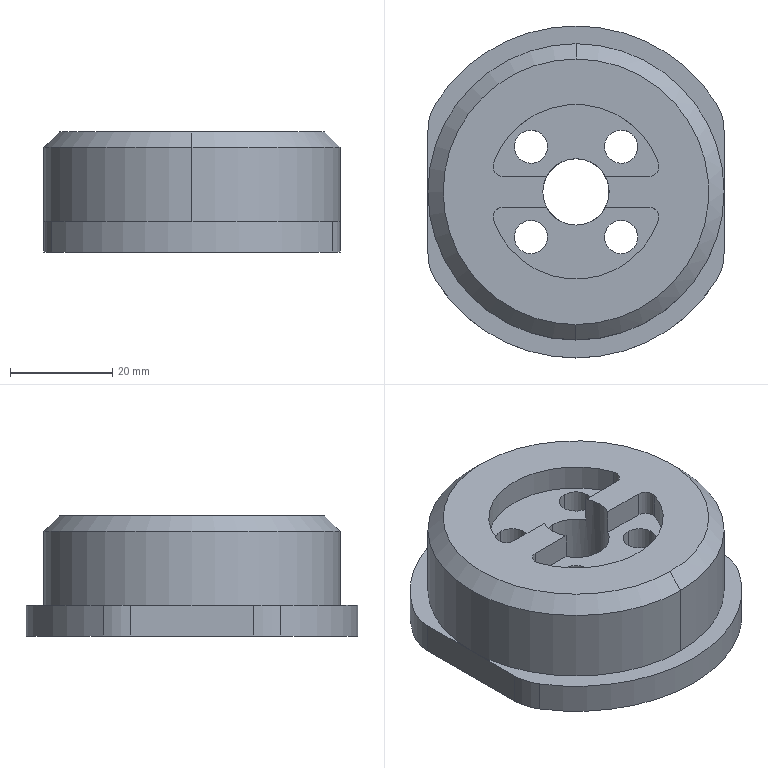CAM job | Mastercam | mm | 9 operations | part box 58 x 65 x 23.5
1. Contour (Ramp) | 9 - 10 平铣刀
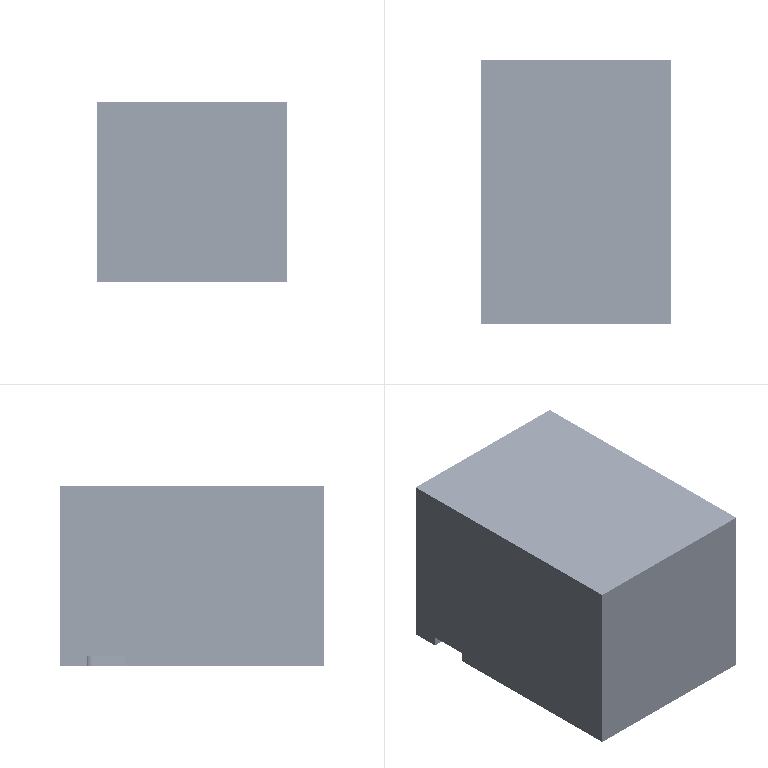2. Contour (2D) | 10 - 10 平铣刀
3. Drill/Counterbore | 7 - 6 倒角刀
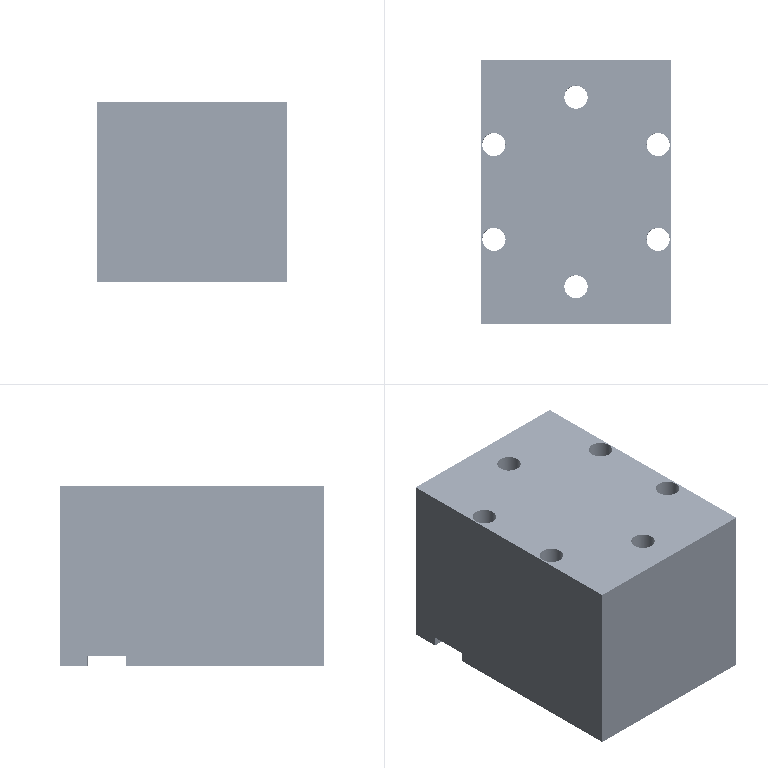4. Contour (Ramp) | 6 - 6 平铣刀
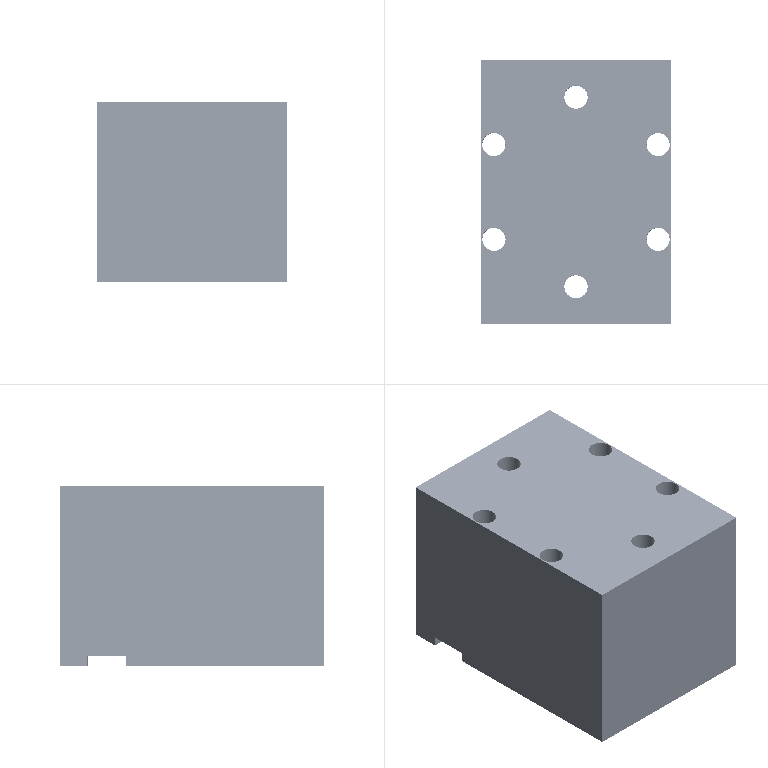5. Contour (Remachining) | 3 - 3 平铣刀
6. 2D High Speed (2D Area Mill) | 3 - 3 平铣刀
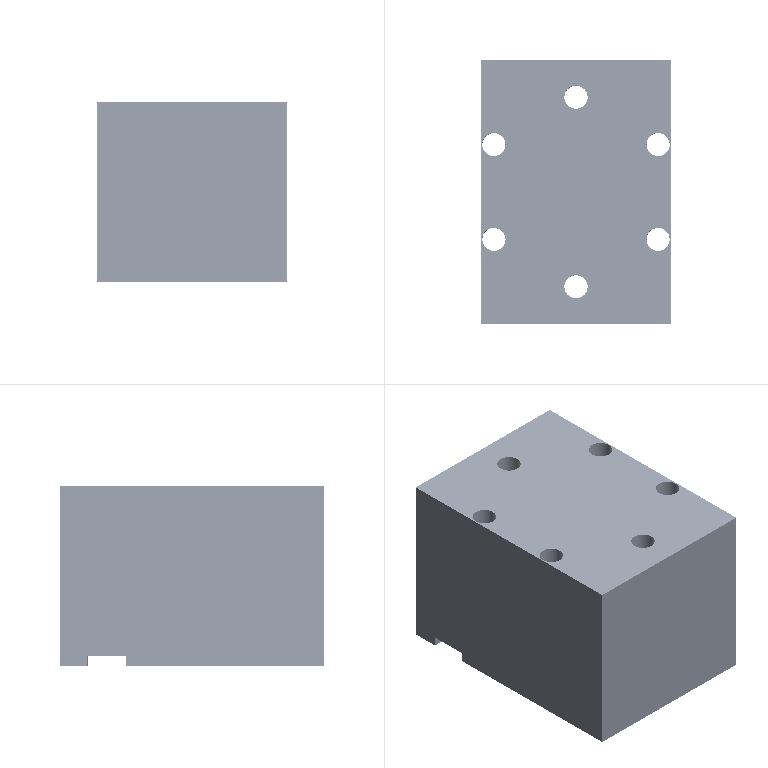7. Contour (Ramp) | 3 - 3 平铣刀
8. Contour (2D chamfer) | 7 - 6 倒角刀
9. Drill/Counterbore | 7 - 6 倒角刀